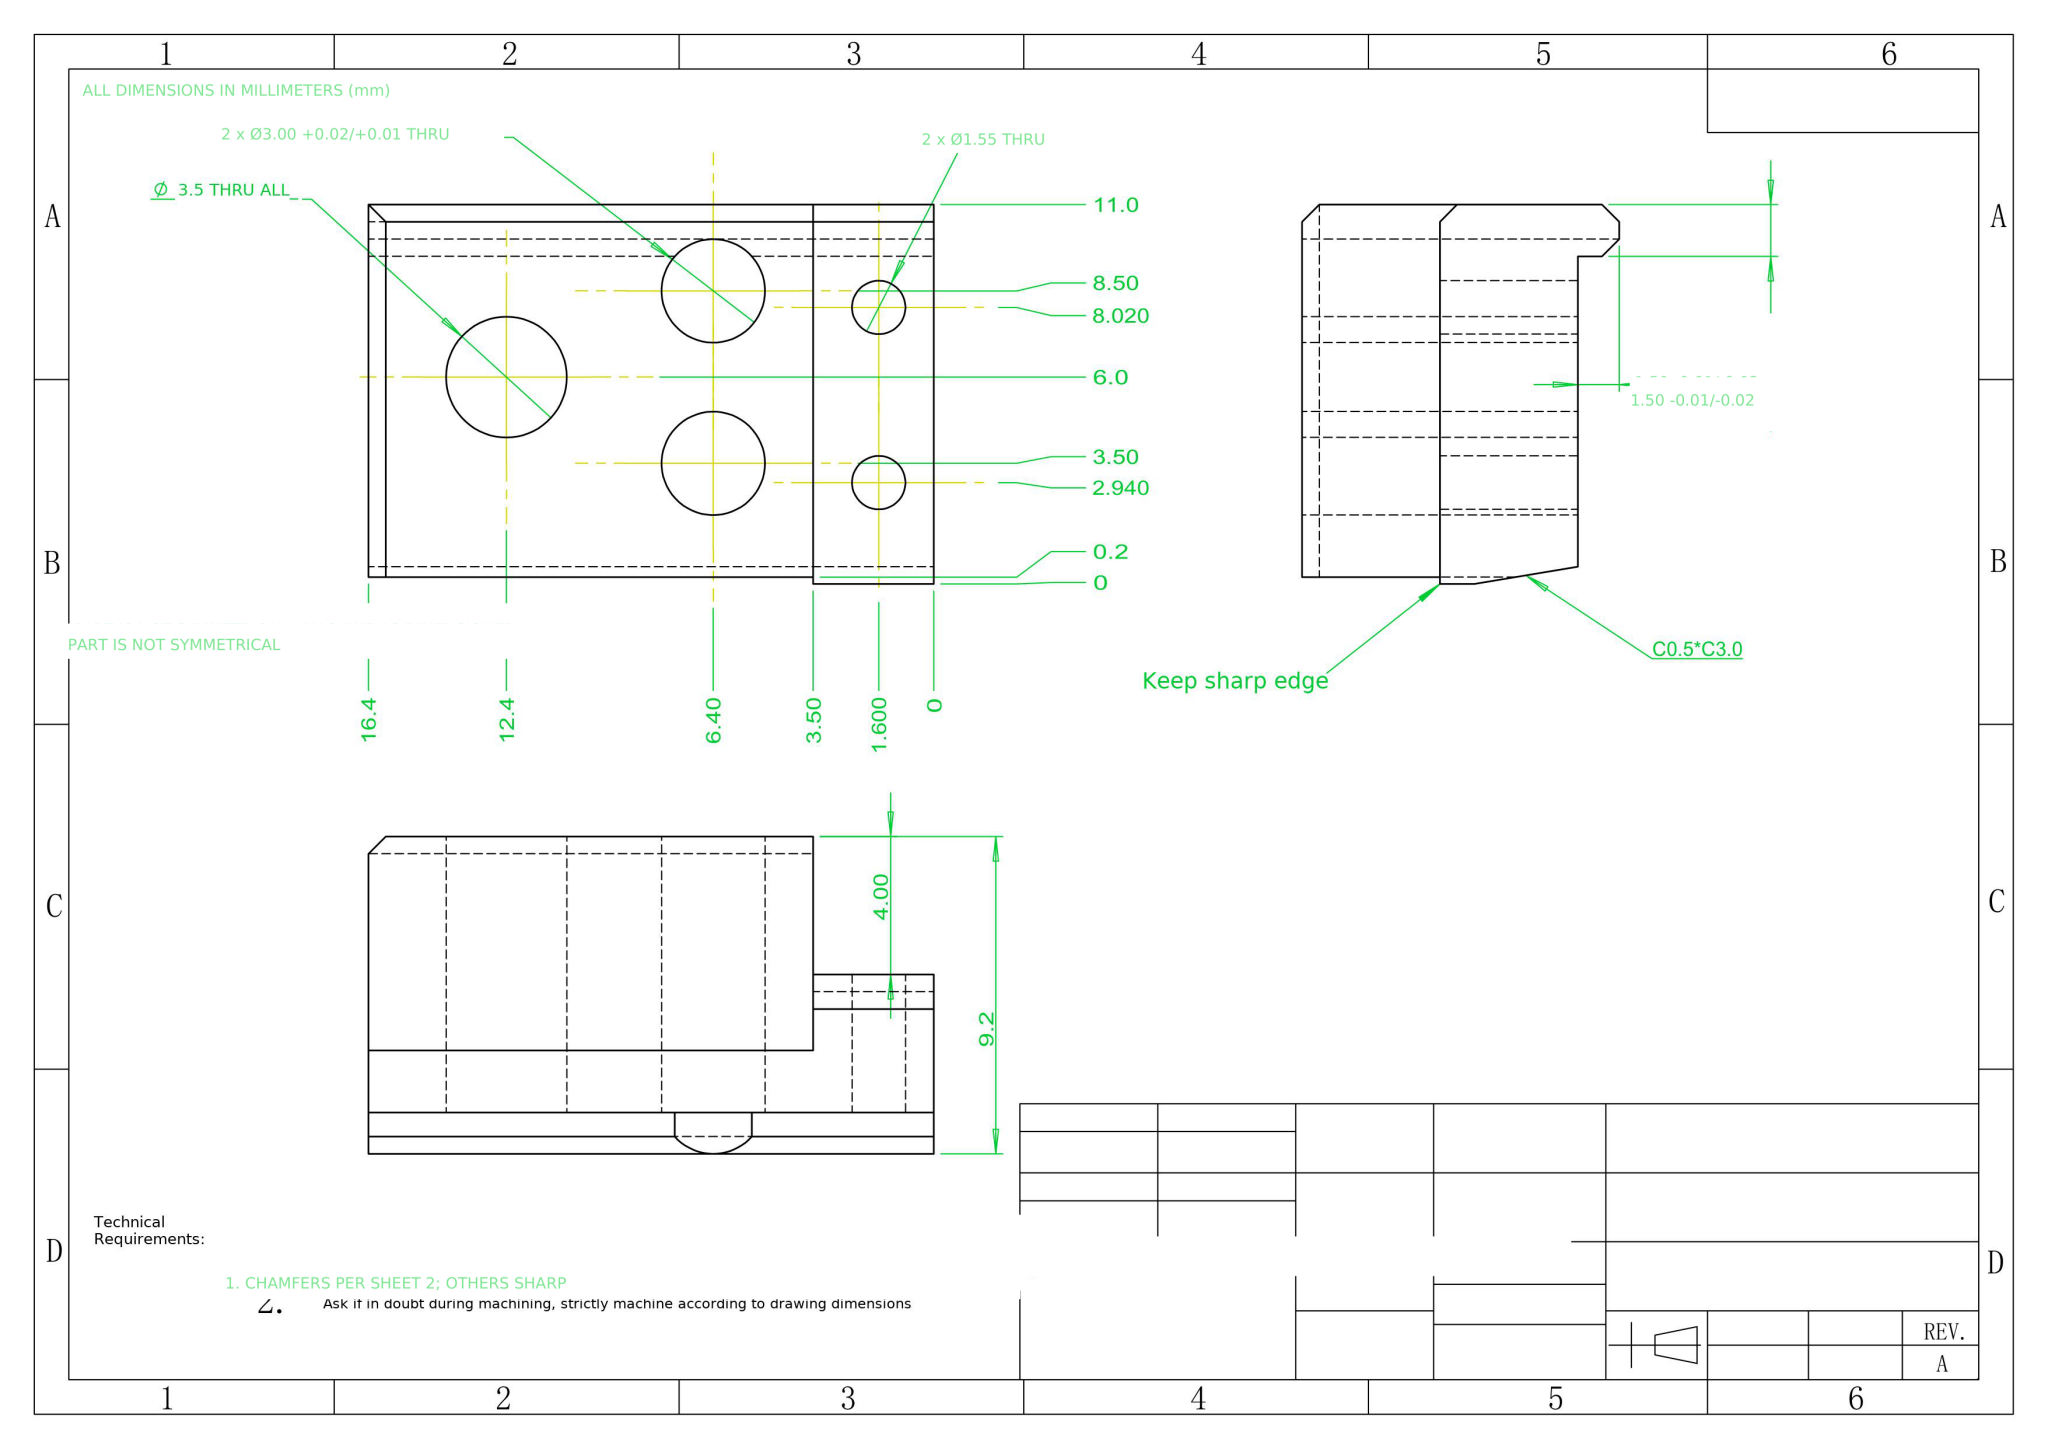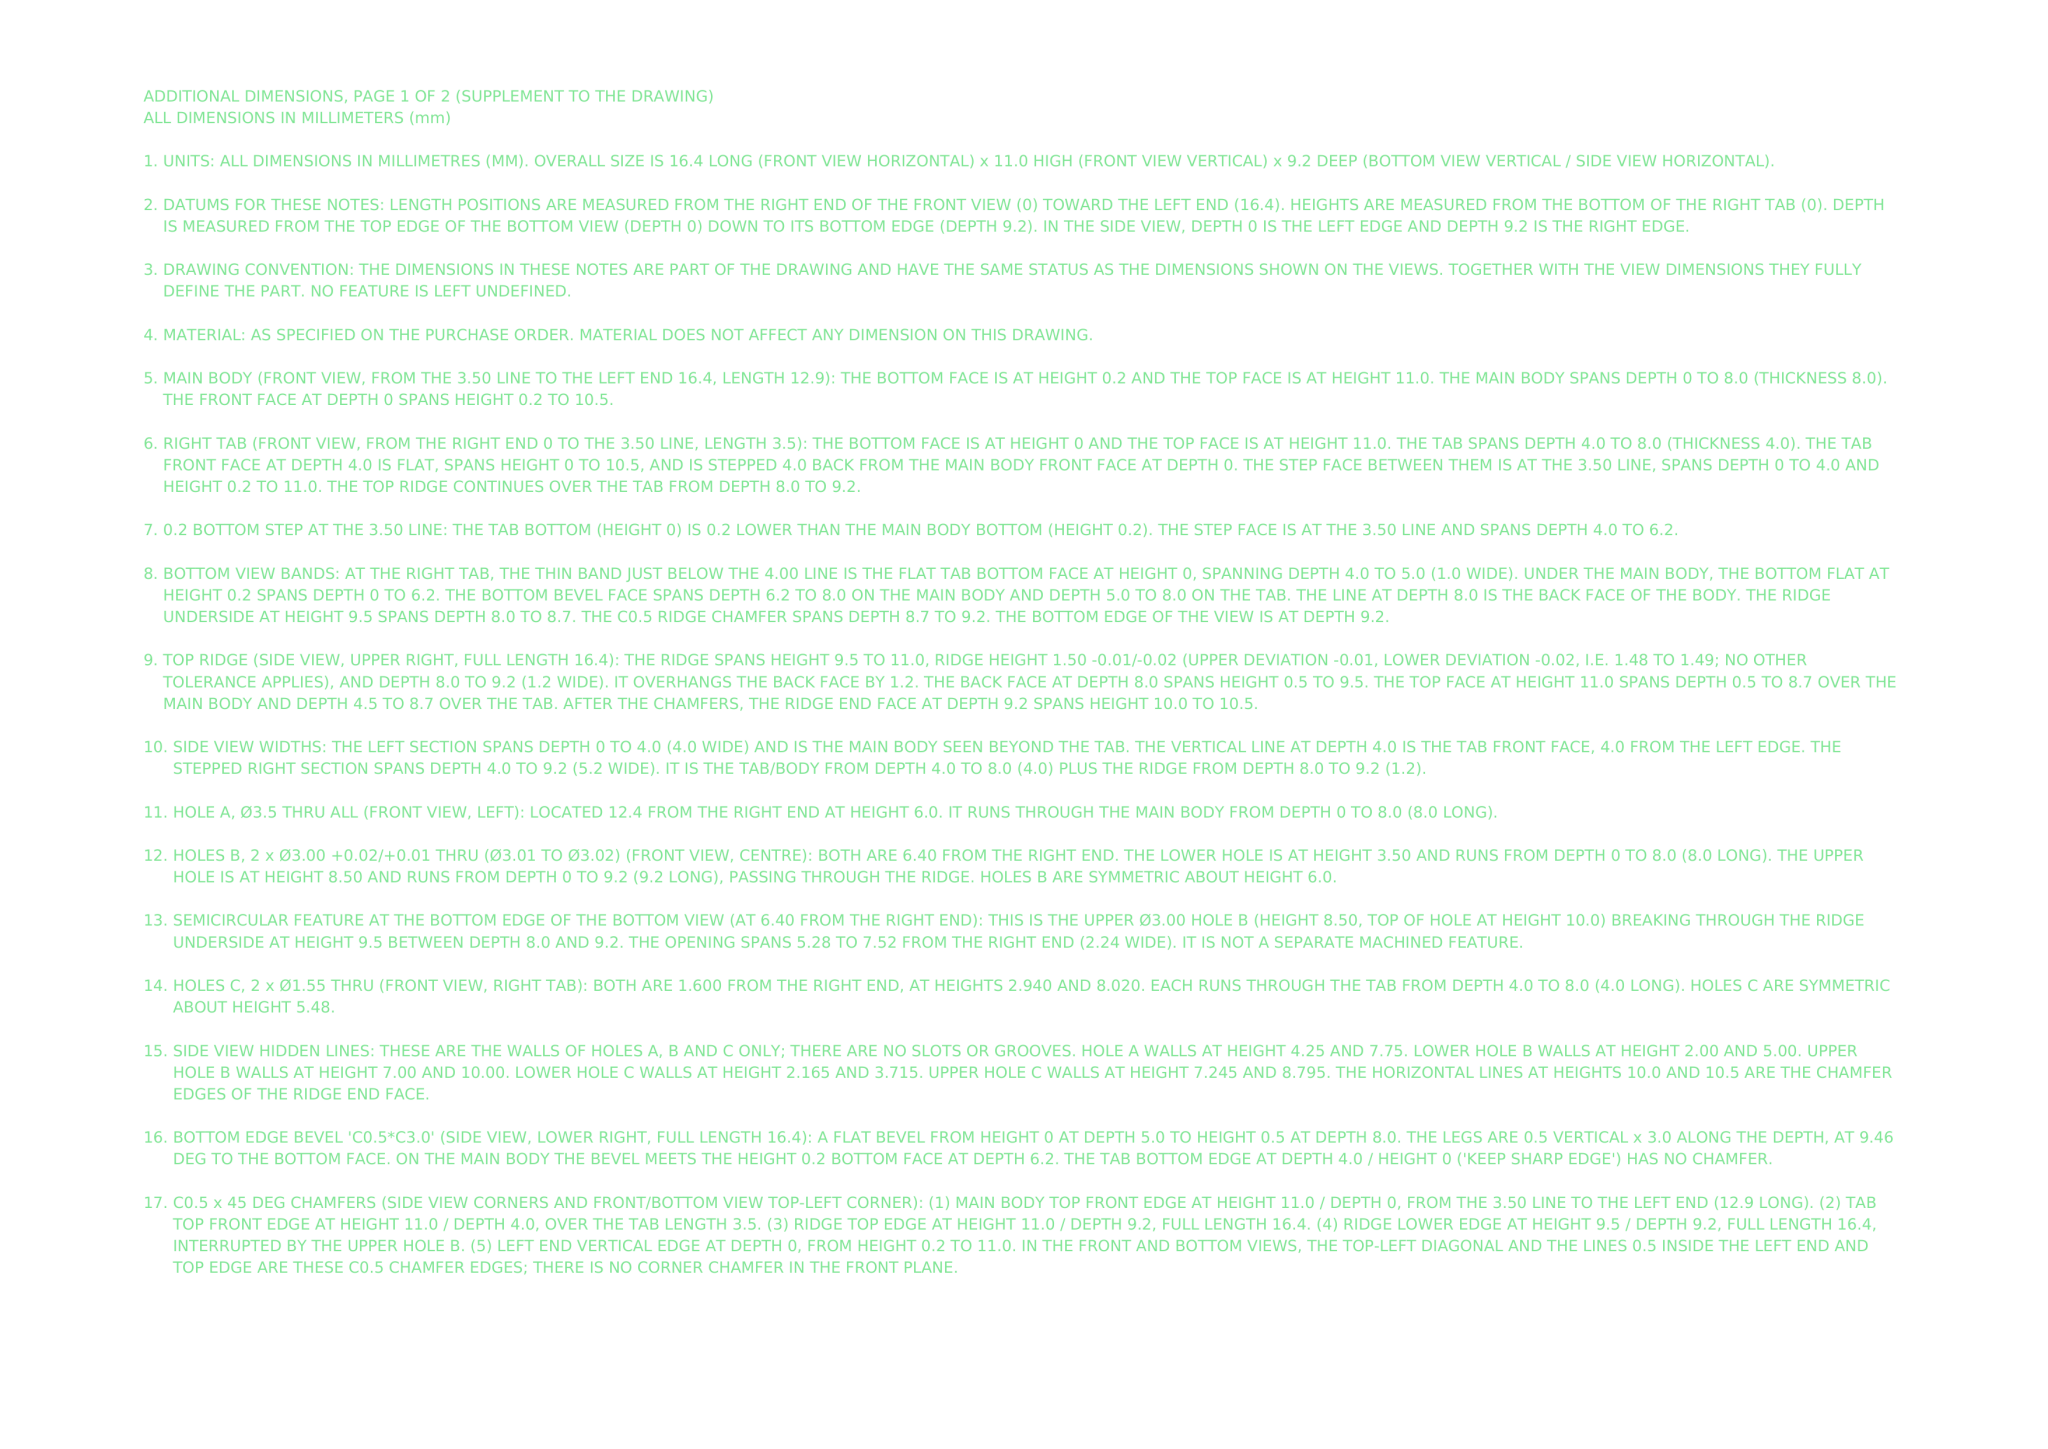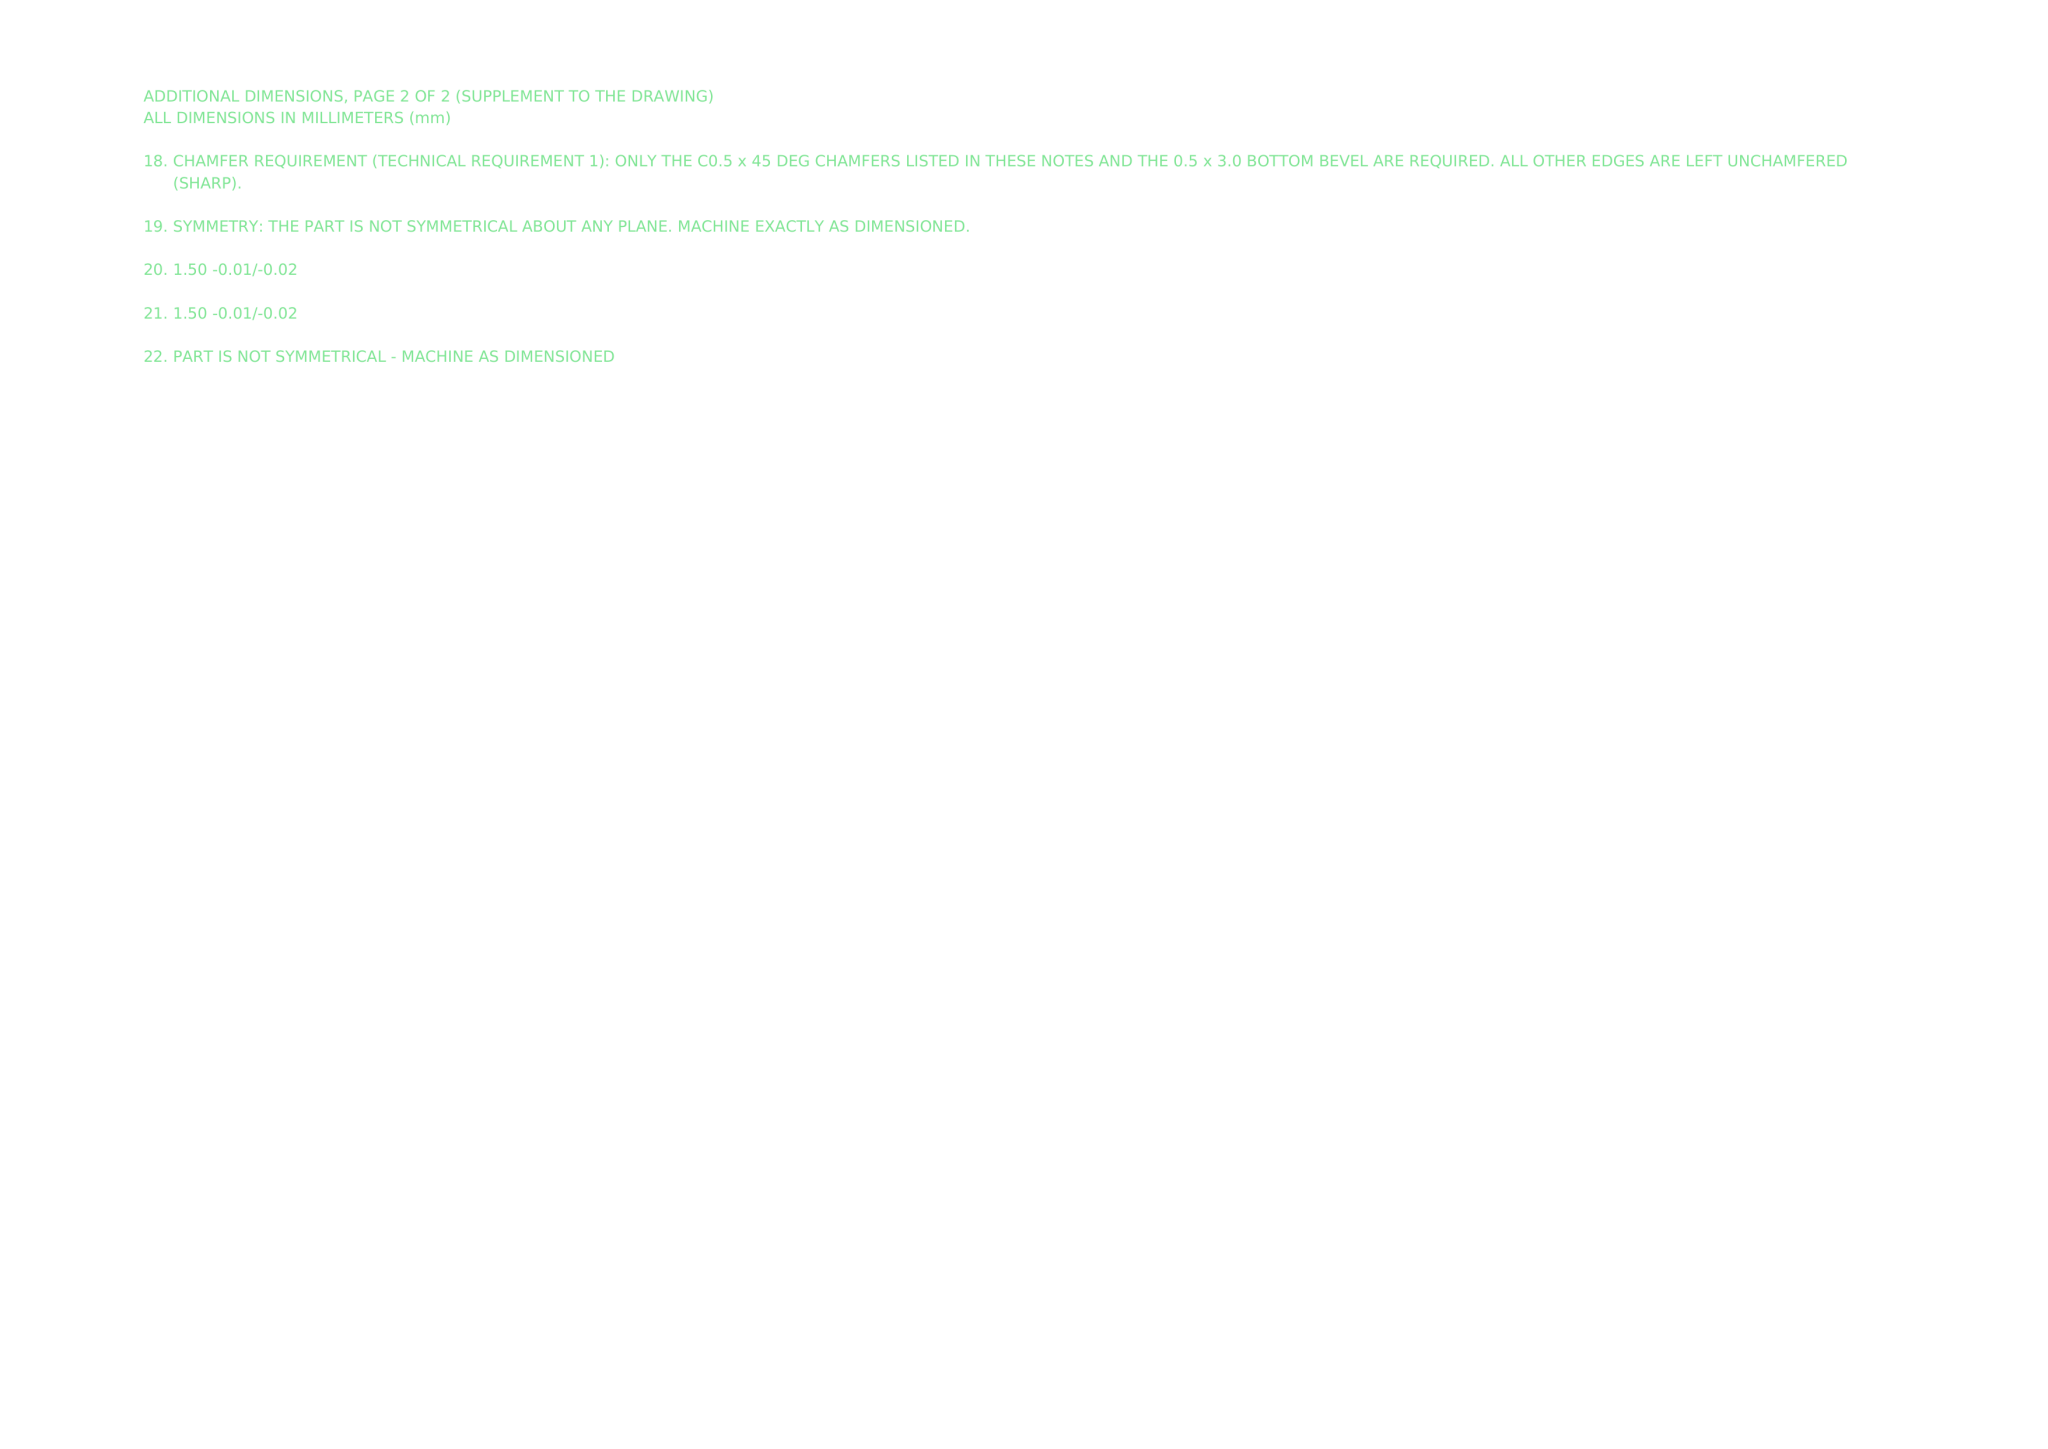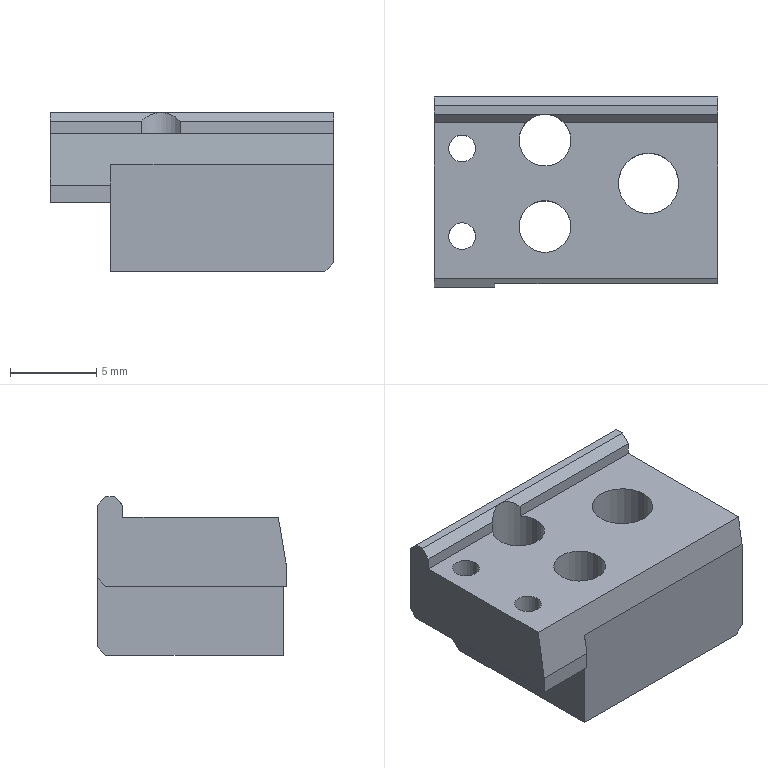Part | NX | mm | 1 solid | 30 faces | box 16.4 x 11 x 9.2 mm | volume 1079 mm3 | plane 20 | cylinder 10 | commonest cylinder face diameters 3 x4 1.55 x4 3.5 x2